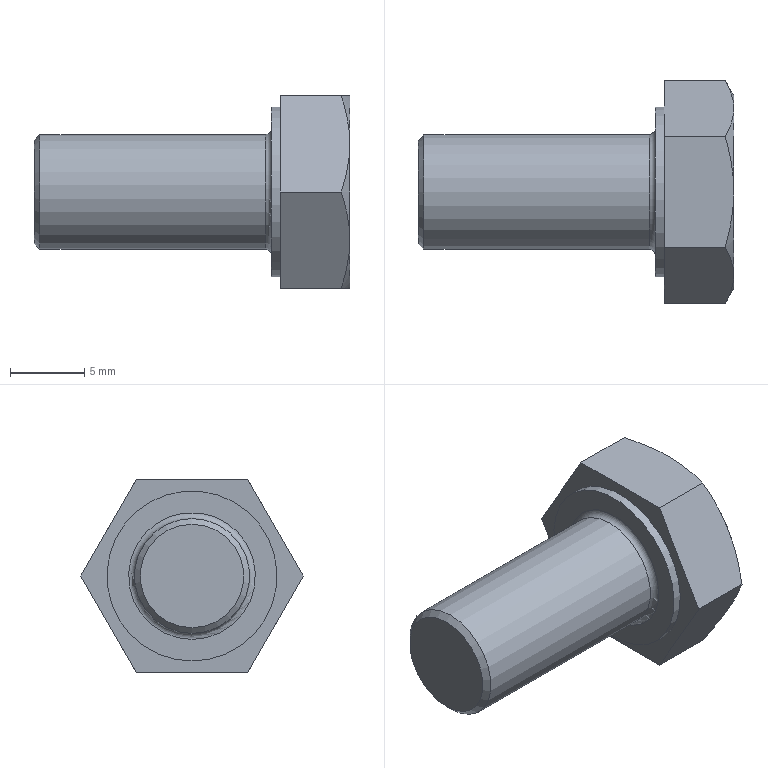Component | NX | GB-T5782-2000_M8X16_2 | 1 solid | 20 faces | volume 1503 mm3 | plane 10 | cone 7 | cylinder 2 | torus 1 | commonest cylinder face diameters 11.47 x1 7.76 x1